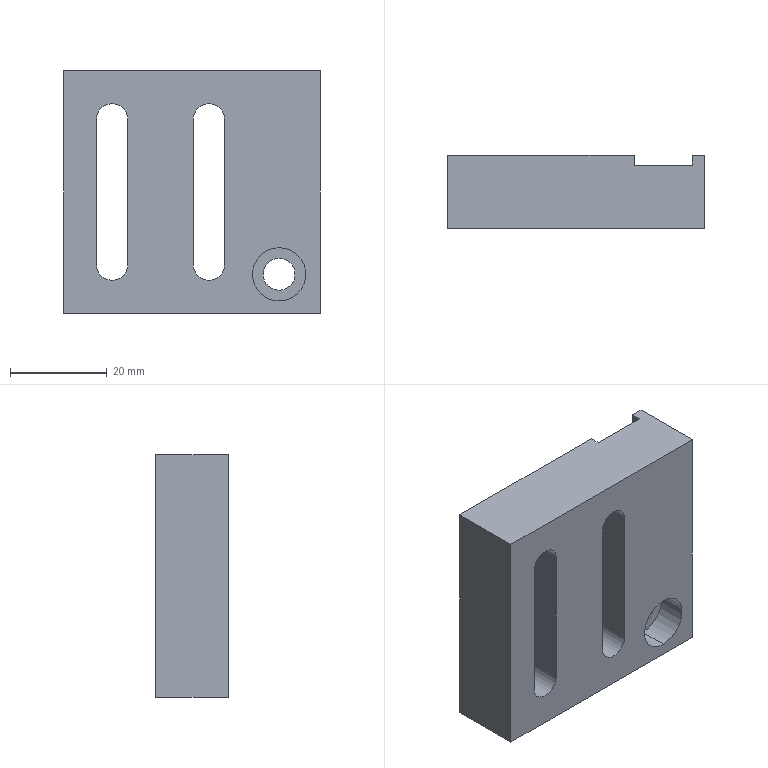Component | SolidWorks | ZL-10-01BasePlate-1 | 1 solid | 23 faces | box 53 x 15 x 50 mm | volume 30895 mm3 | plane 15 | cylinder 8 | commonest cylinder face diameters 6.5 x4 11 x2 6.6 x2
build123d program:
from build123d import *

# Parameters (mm, degrees)
SKETCH1_W                                       = 53
SKETCH1_H                                       = 15
EXTRUDE1_DEPTH                                  = 25
SKETCH2_W                                       = 12
SKETCH2_H                                       = 2
CUT_EXTRUDE1_DEPTH                              = 59.543
CUT_EXTRUDE2_DEPTH                              = 40.399
LPATTERN1_COUNT                                 = 2
LPATTERN1_PITCH                                 = 20
M6_HEX_SOCKET_HEAD_CAP_SCREW_CBORE1_D           = 6.6
M6_HEX_SOCKET_HEAD_CAP_SCREW_CBORE1_CBORE_D     = 11
M6_HEX_SOCKET_HEAD_CAP_SCREW_CBORE1_CBORE_DEPTH = 6


with BuildPart() as part:
    # Sketch1 → Extrude1 (new, symmetric)
    with BuildSketch(Plane.XY):
        with Locations((0, 7.5)):
            Rectangle(SKETCH1_W, SKETCH1_H)
    extrude(amount=EXTRUDE1_DEPTH, both=True)

    # Sketch2 → Cut-Extrude1 (cut, through all)
    with BuildSketch(Plane.XY.offset(25)):
        with Locations((18, 14)):
            Rectangle(SKETCH2_W, SKETCH2_H)
    extrude(amount=-CUT_EXTRUDE1_DEPTH, mode=Mode.SUBTRACT)

    # Sketch3 → Cut-Extrude2 (cut, through all)
    with BuildSketch(Plane(origin=(0, 15, 0), x_dir=(1, 0, 0), z_dir=(0, 1, 0))):
        with BuildLine():
            Line((-19.75, 15), (-19.75, -15))
            ThreePointArc((-19.75, -15), (-16.5, -18.25), (-13.25, -15))
            Line((-13.25, -15), (-13.25, 15))
            ThreePointArc((-13.25, 15), (-16.5, 18.25), (-19.75, 15))
        make_face()
    cut_extrude2 = extrude(amount=-CUT_EXTRUDE2_DEPTH, mode=Mode.SUBTRACT)

    # LPattern1: Cut-Extrude2 ×2
    with Locations(*[(i * LPATTERN1_PITCH, 0, 0) for i in range(1, LPATTERN1_COUNT)]):
        add(cut_extrude2, mode=Mode.SUBTRACT)

    # M6 Hex Socket Head Cap Screw CBORE1 (through all)
    with Locations(Plane(origin=(1.735, 0, -20.386), x_dir=(-1, 0, 0), z_dir=(0, -1, 0))):
        with Locations((-16.265, -3.386)):
            CounterBoreHole(M6_HEX_SOCKET_HEAD_CAP_SCREW_CBORE1_D / 2, M6_HEX_SOCKET_HEAD_CAP_SCREW_CBORE1_CBORE_D / 2, M6_HEX_SOCKET_HEAD_CAP_SCREW_CBORE1_CBORE_DEPTH)


solid = part.part

# Placed as in the assembly
solid = solid.moved(Location((0.8234, -6.251, 0), (0, 0, 0)))